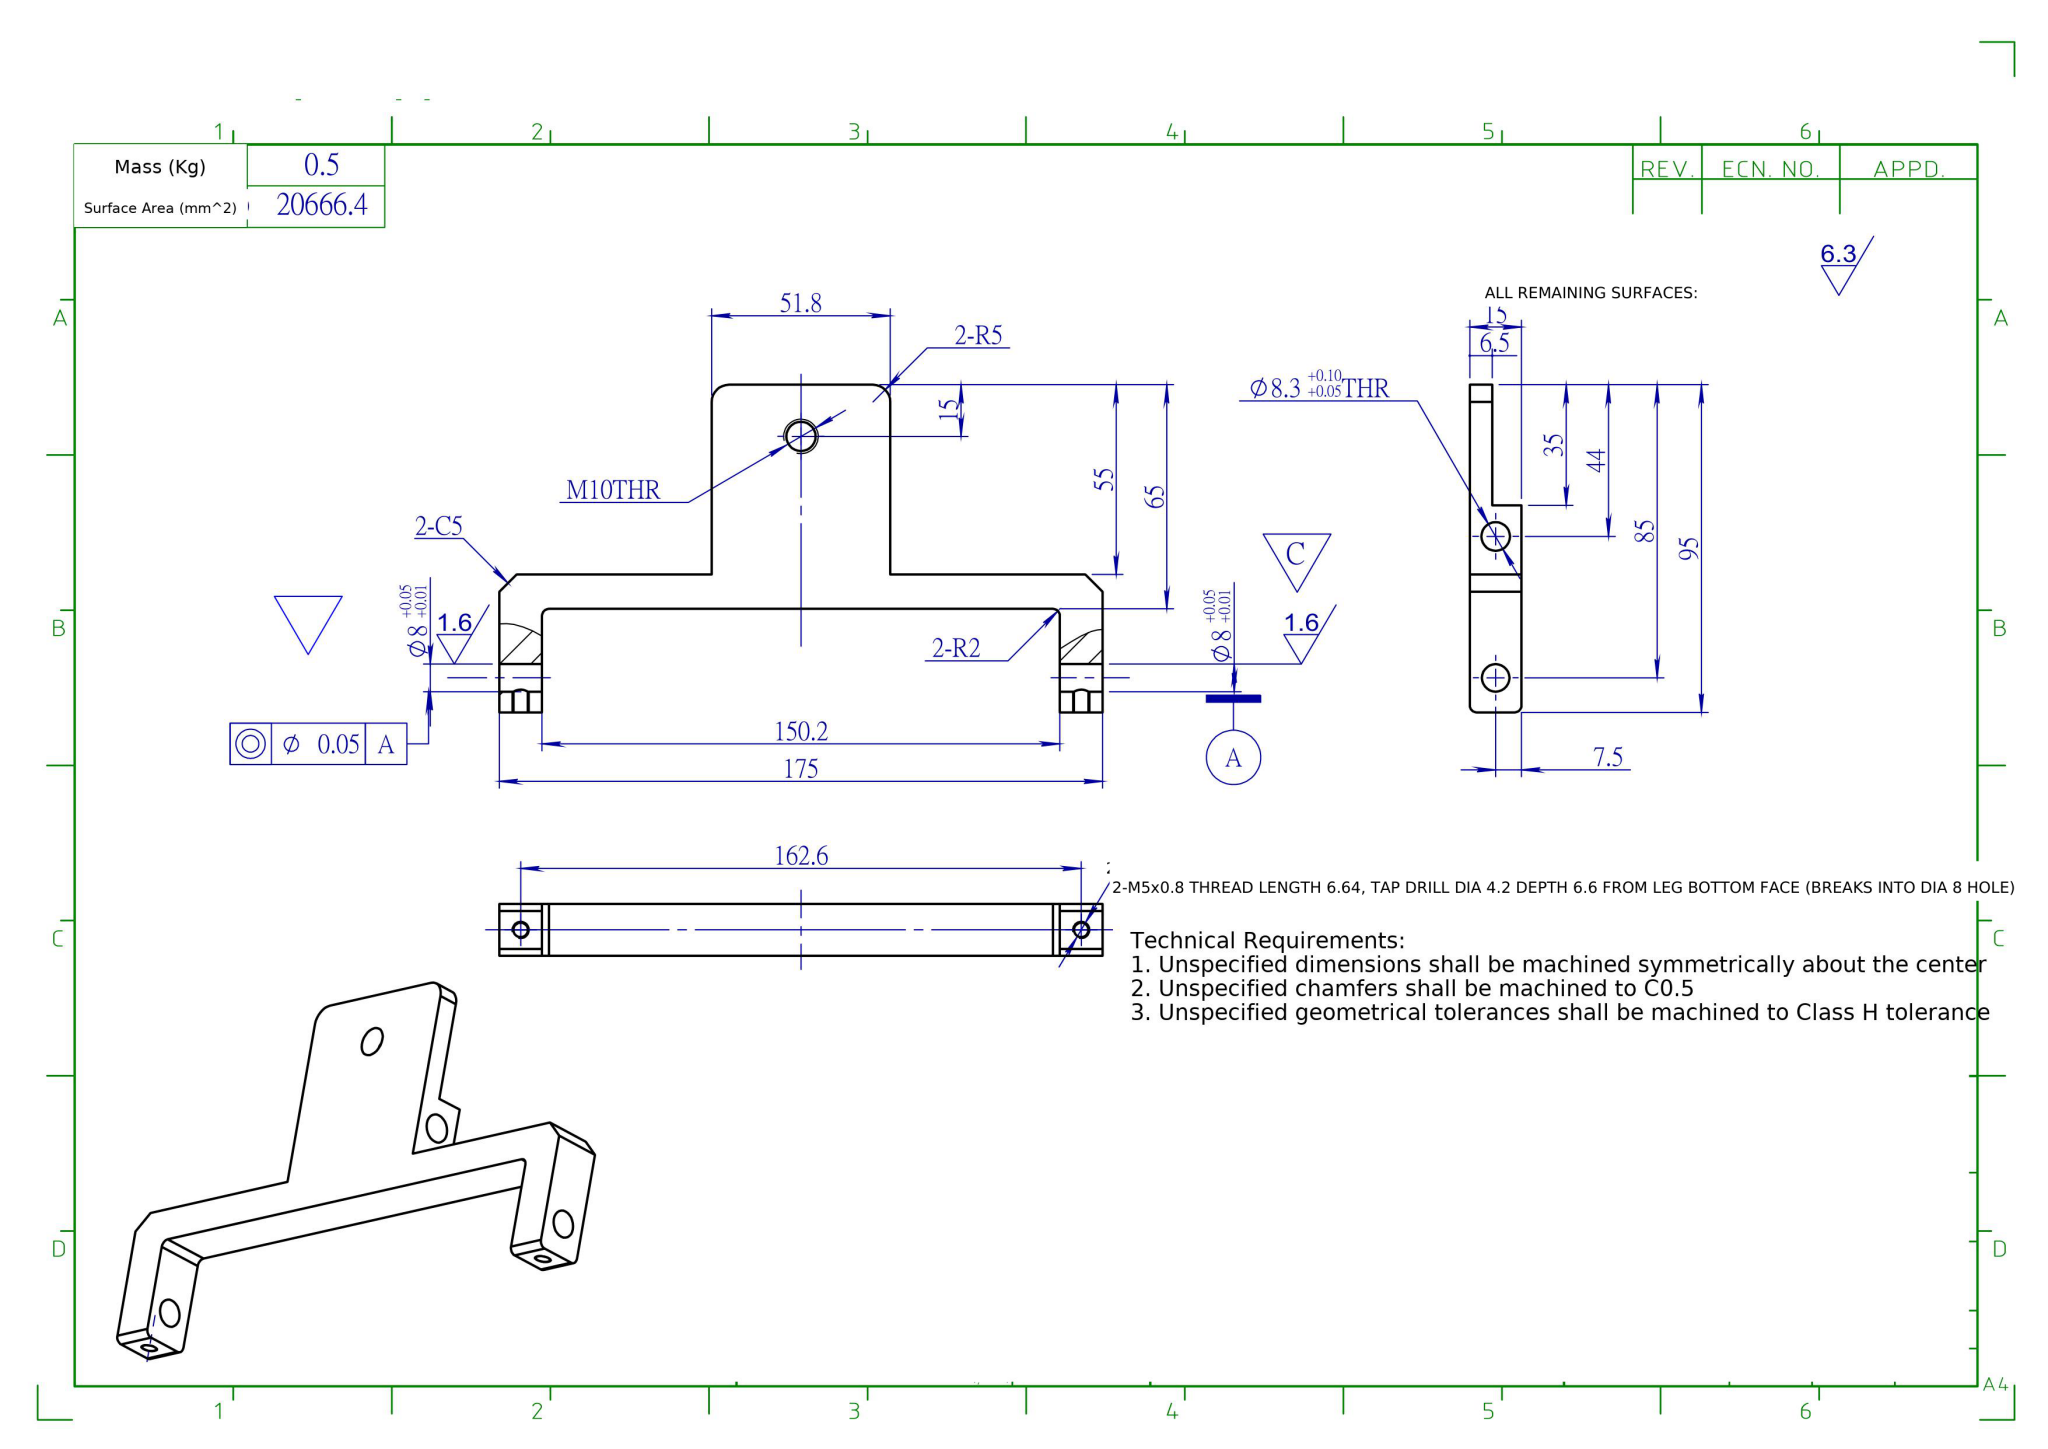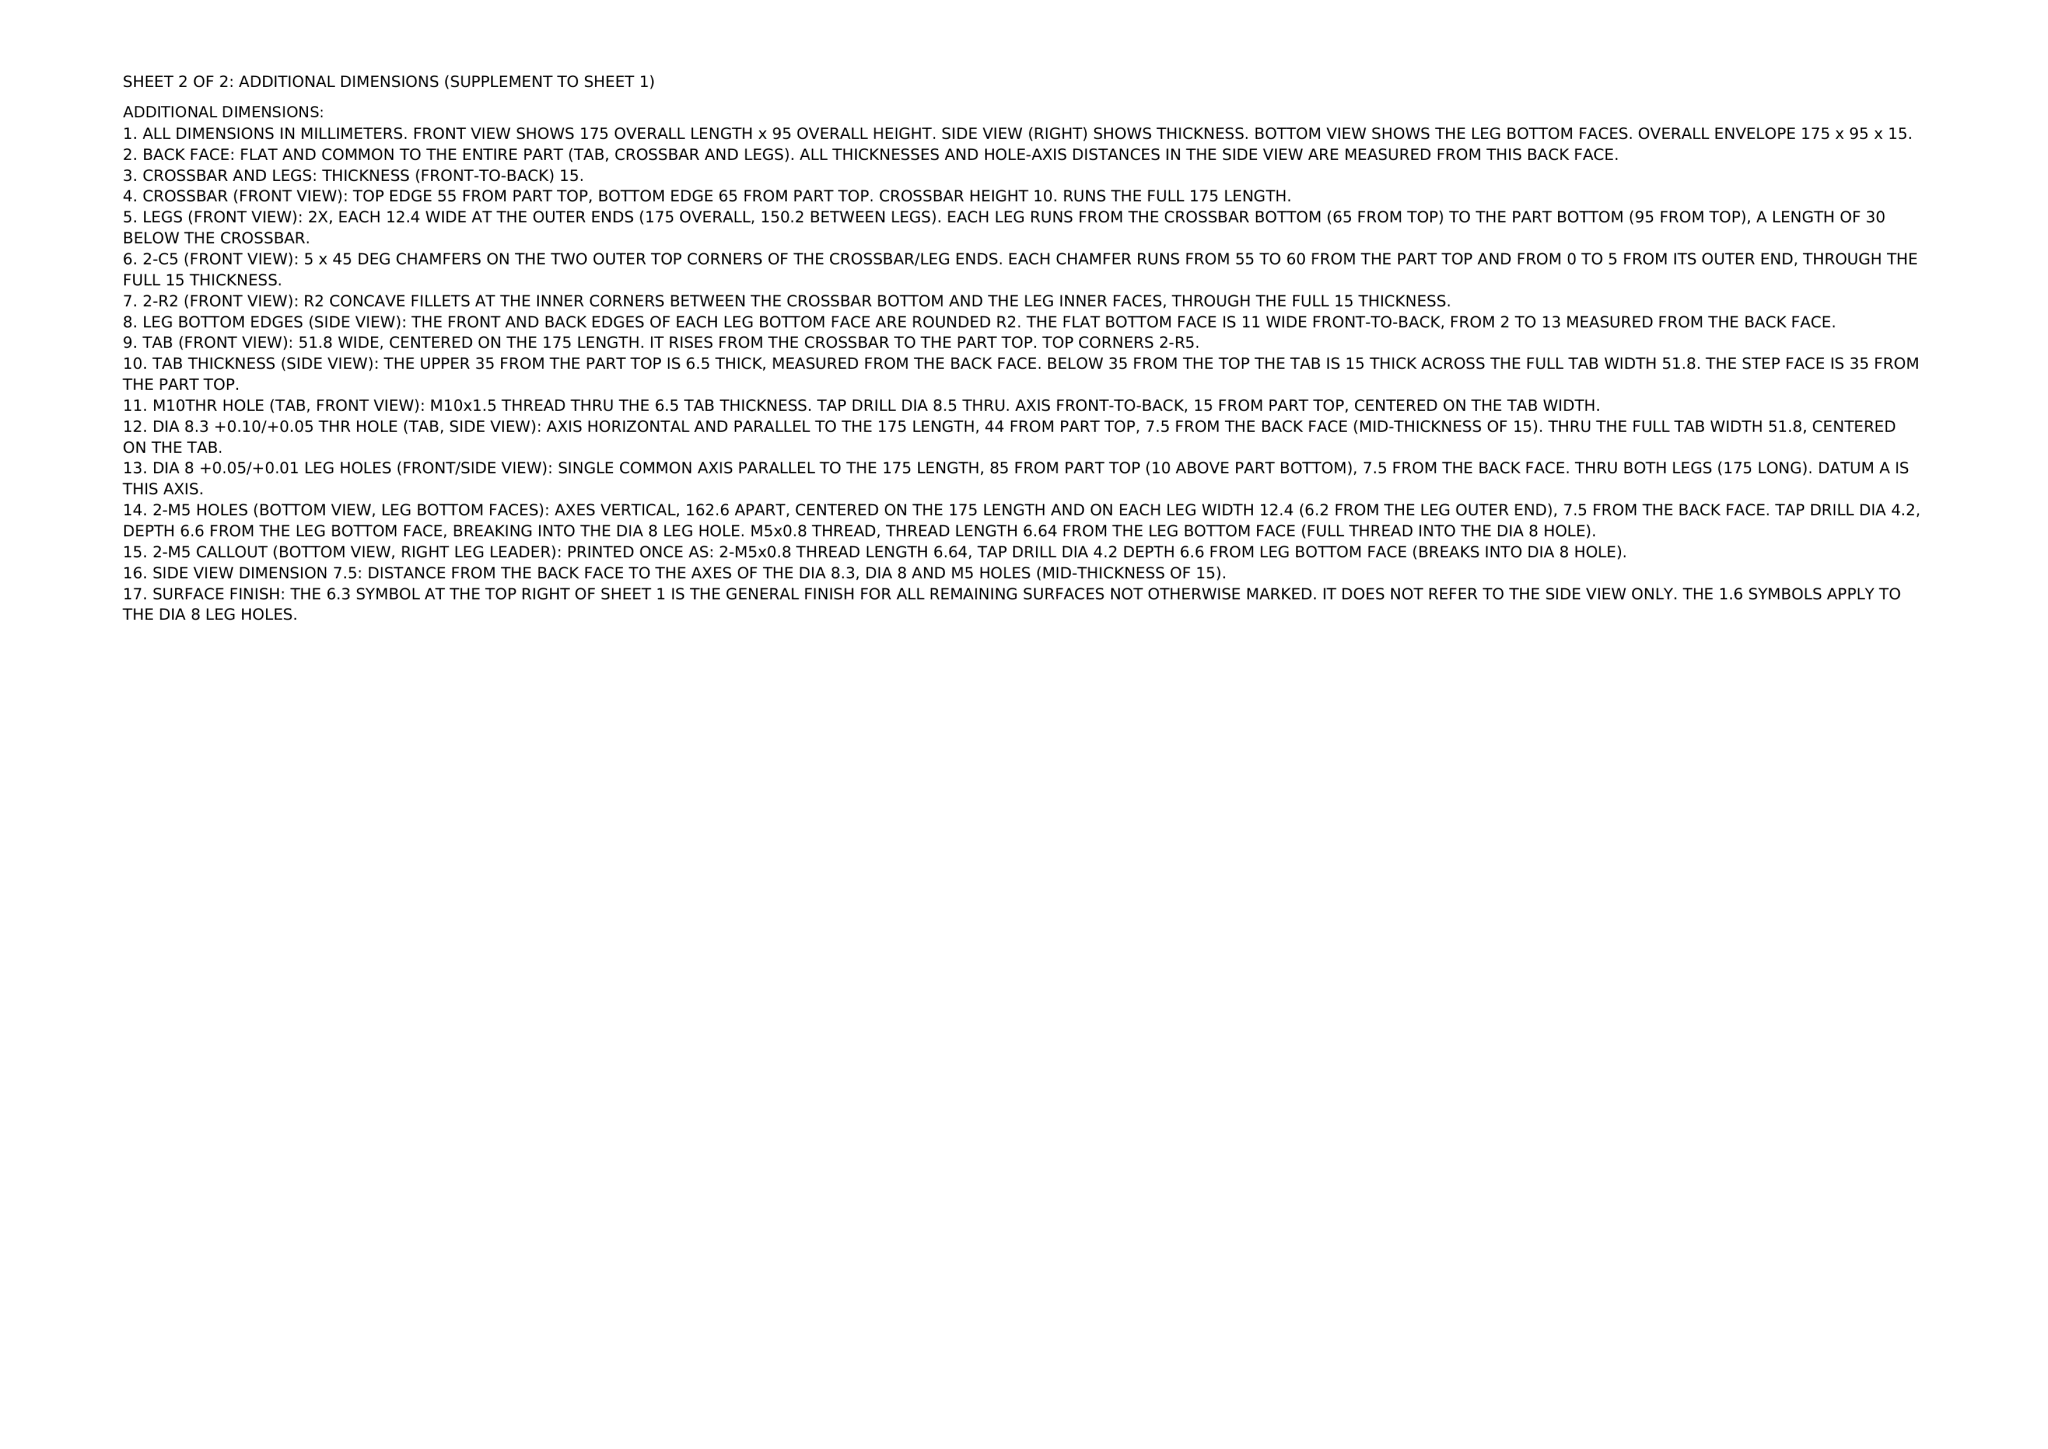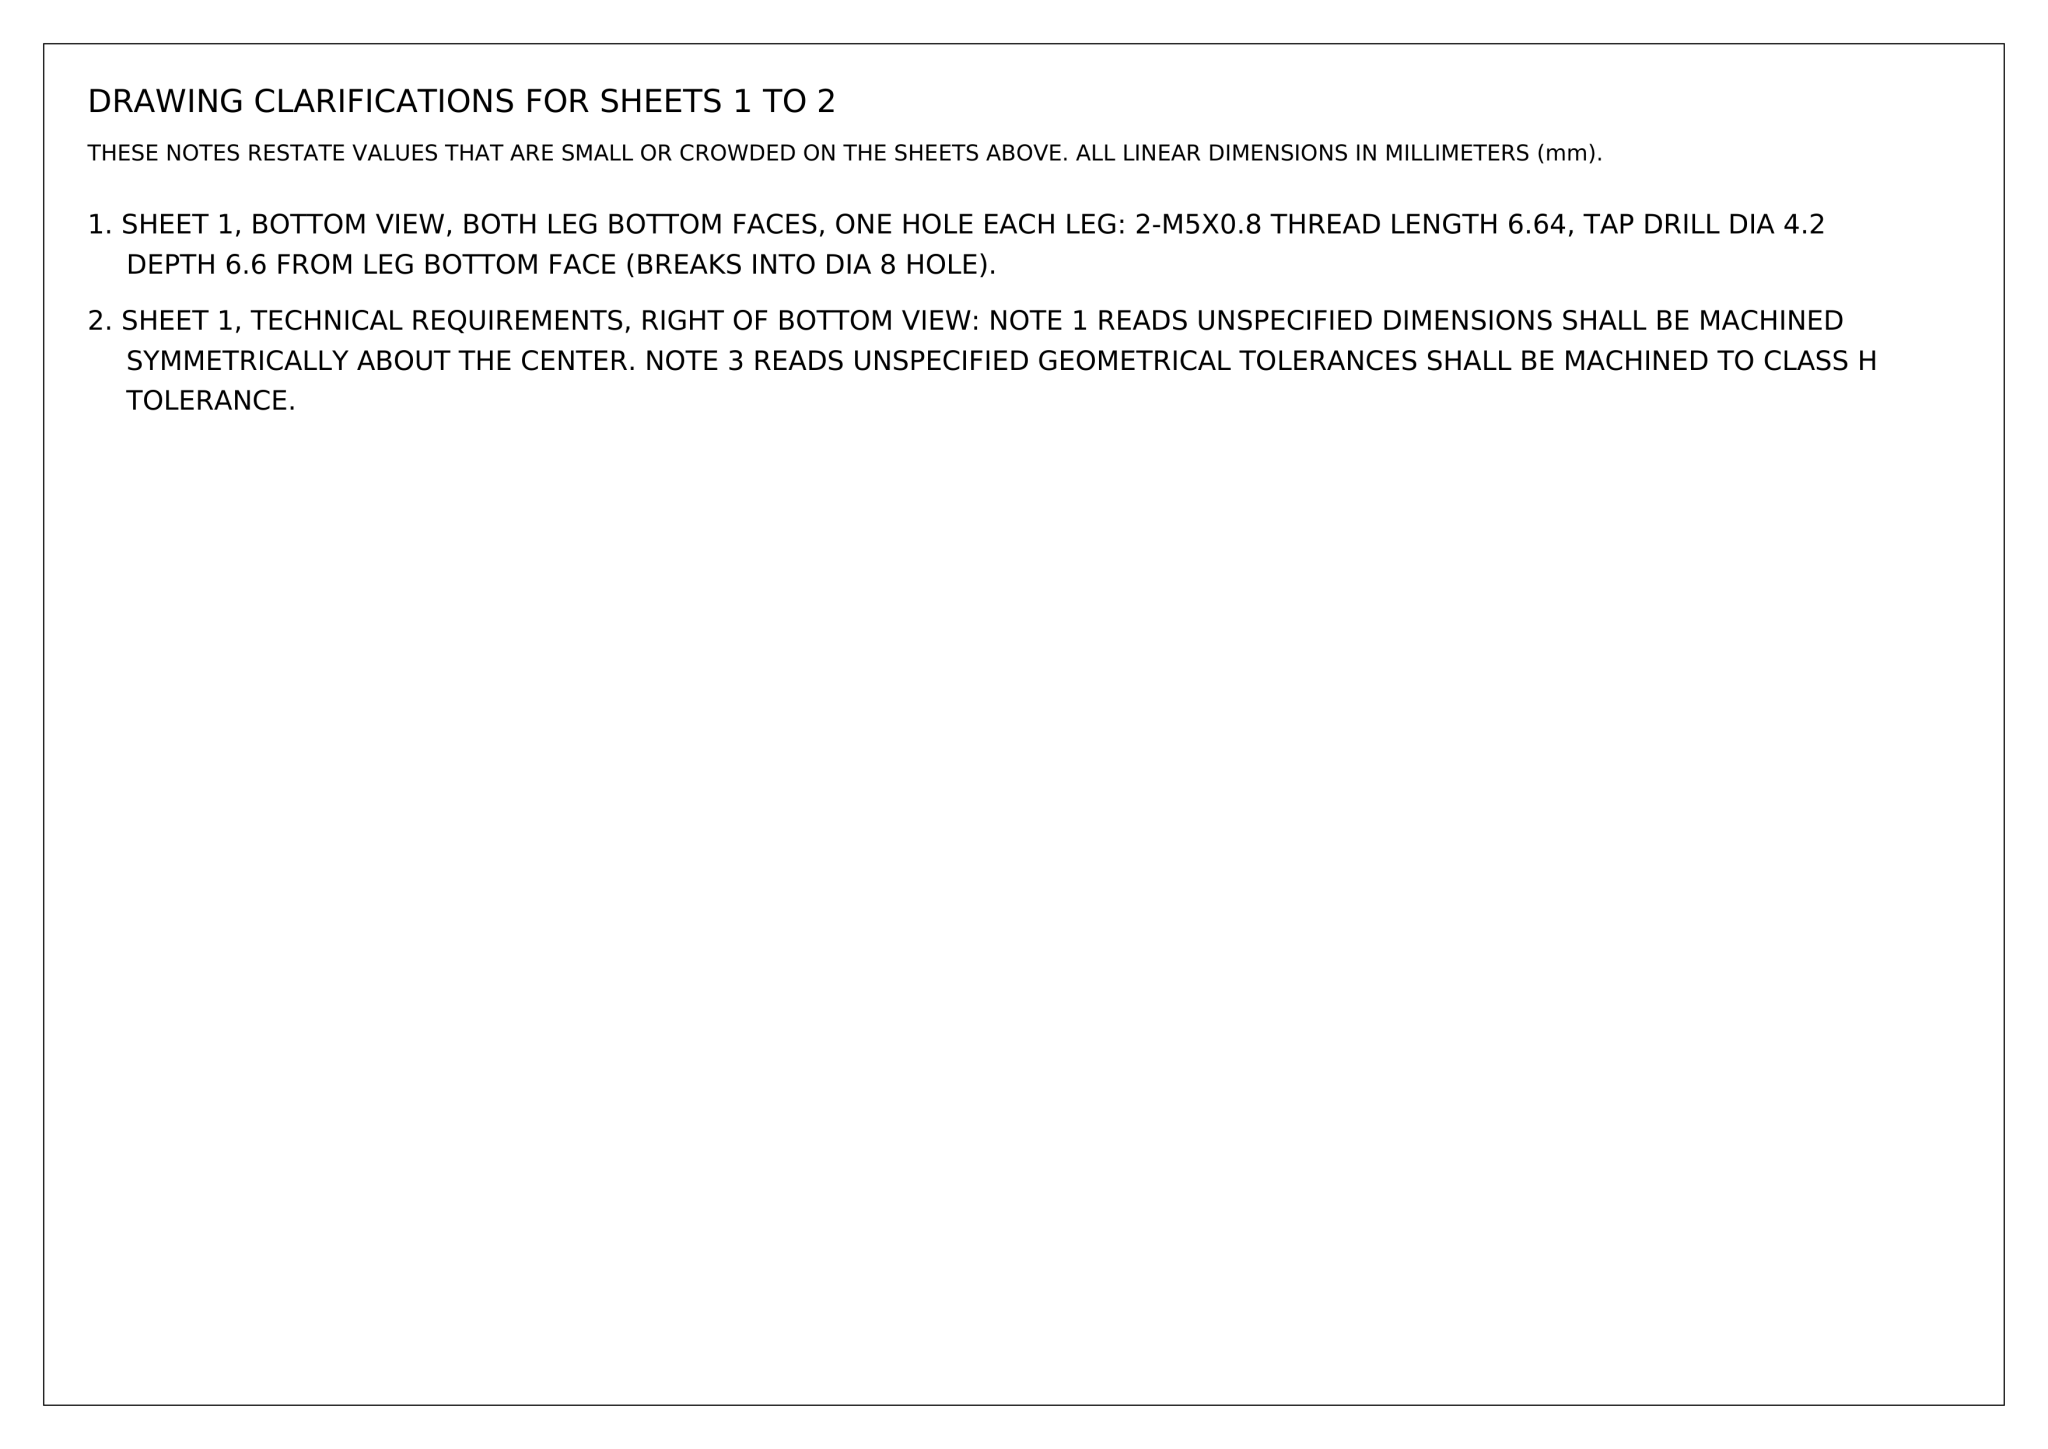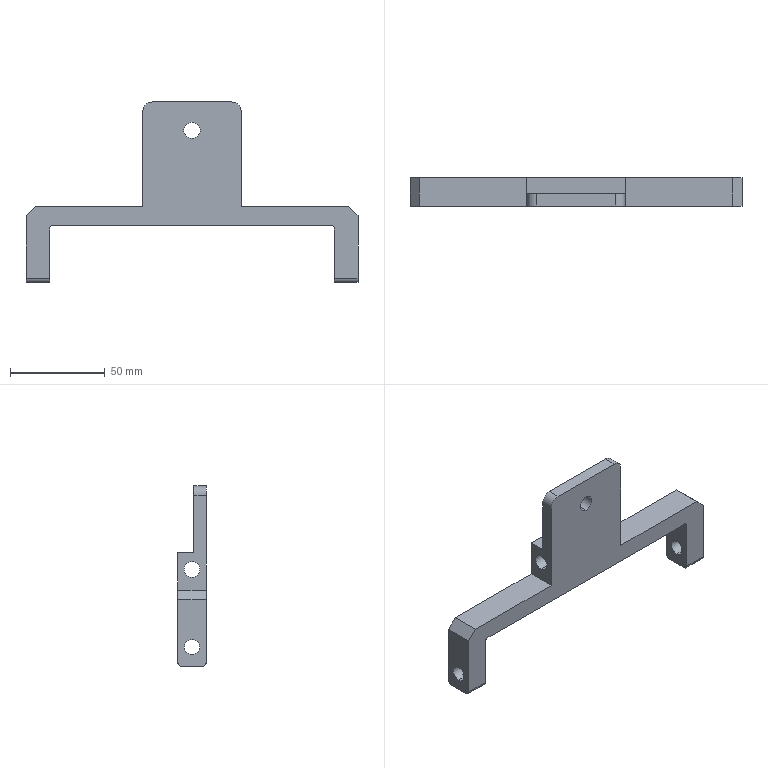Part | NX | mm | 1 solid | 38 faces | box 175 x 15 x 95 mm | volume 59685 mm3 | cylinder 20 | plane 18 | commonest cylinder face diameters 4 x6 4.2 x4 8 x4 8.3 x2 8.5 x2 10 x2